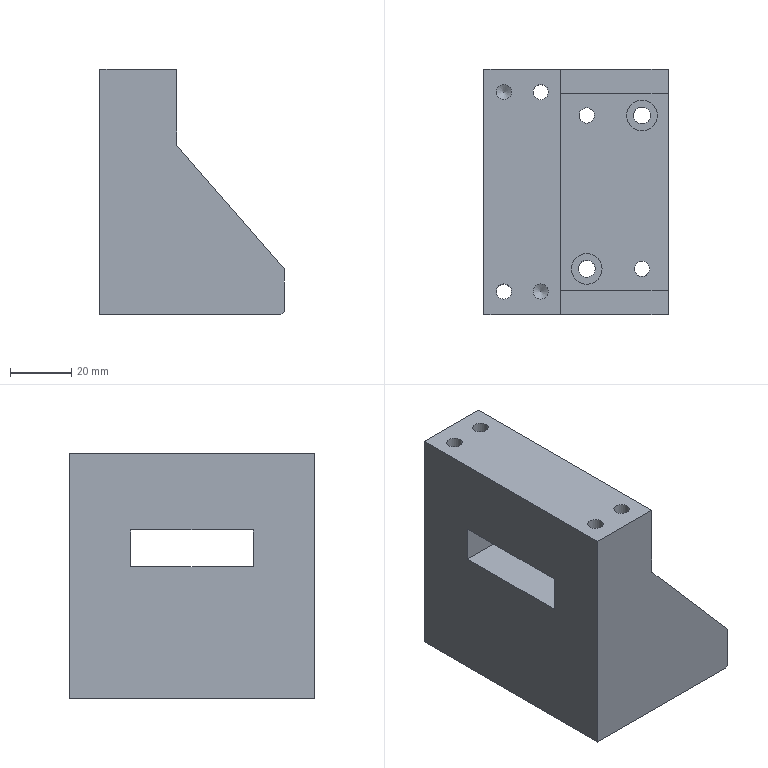Component | NX | DRILL_JIG_SUPPORT | 1 solid | 39 faces | volume 194745 mm3 | plane 19 | cylinder 14 | cone 6 | commonest cylinder face diameters 5 x10 5.5 x2 10 x2